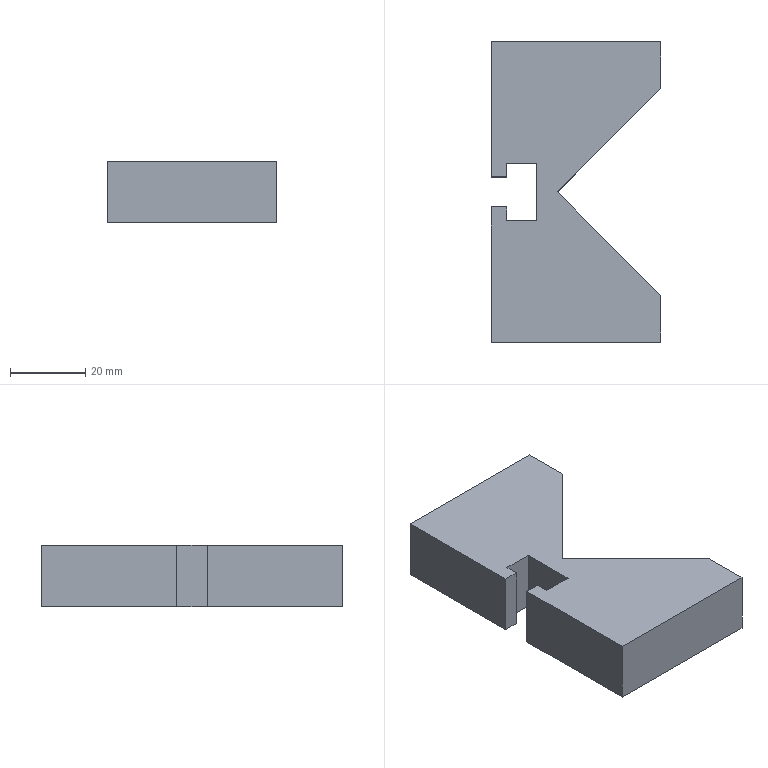Component | NX | V_BLOCK_2 | 1 solid | 17 faces | volume 44414 mm3 | plane 17